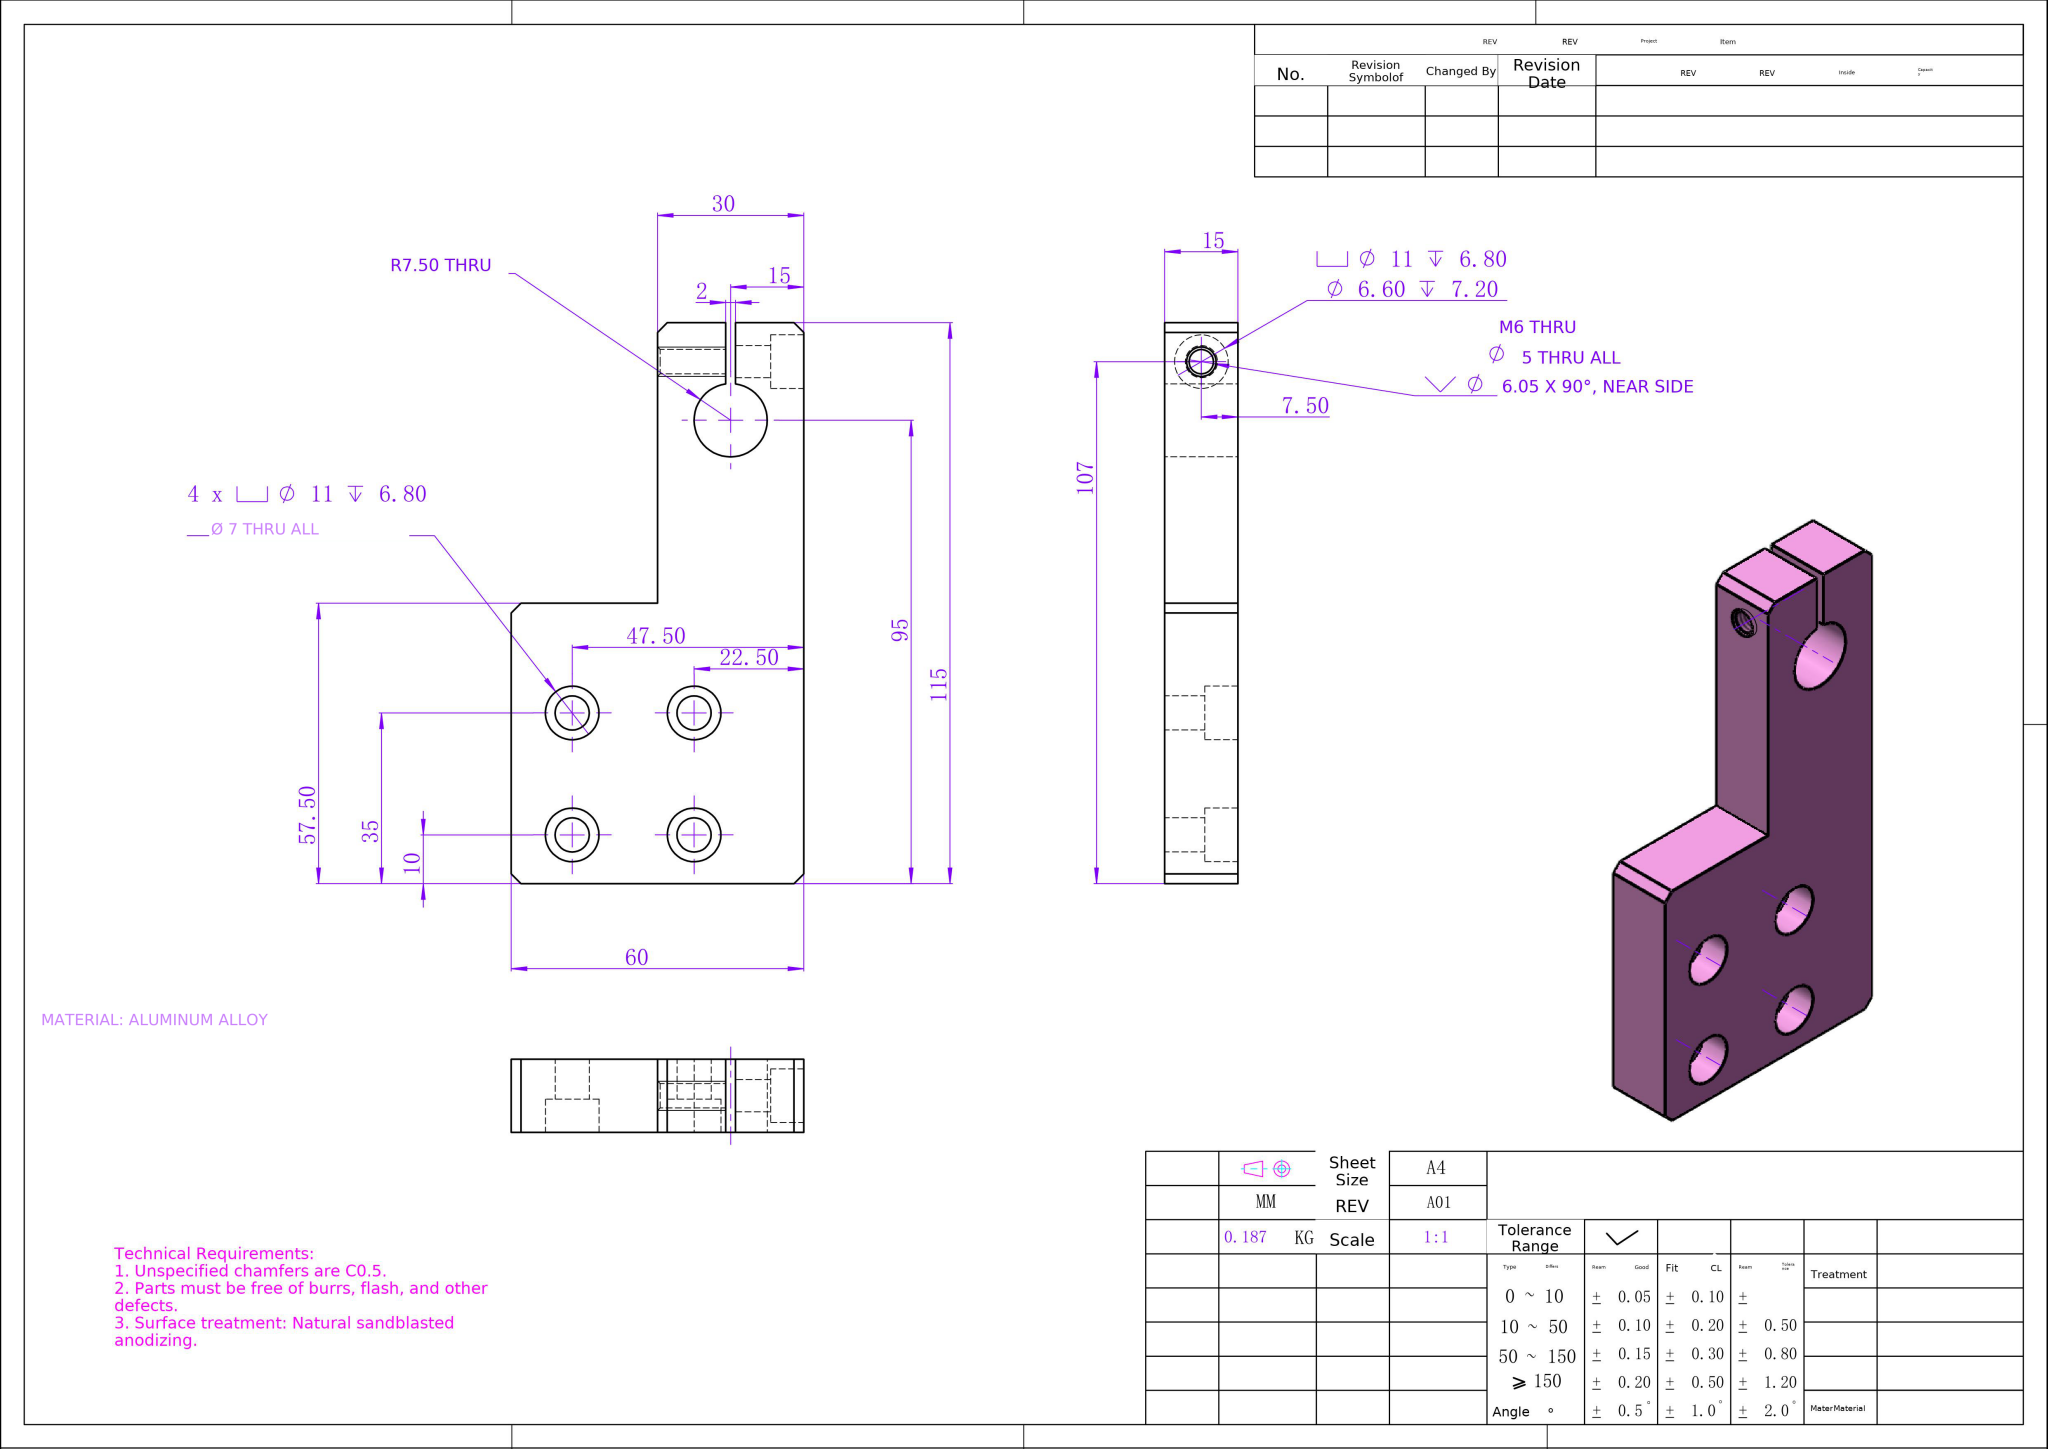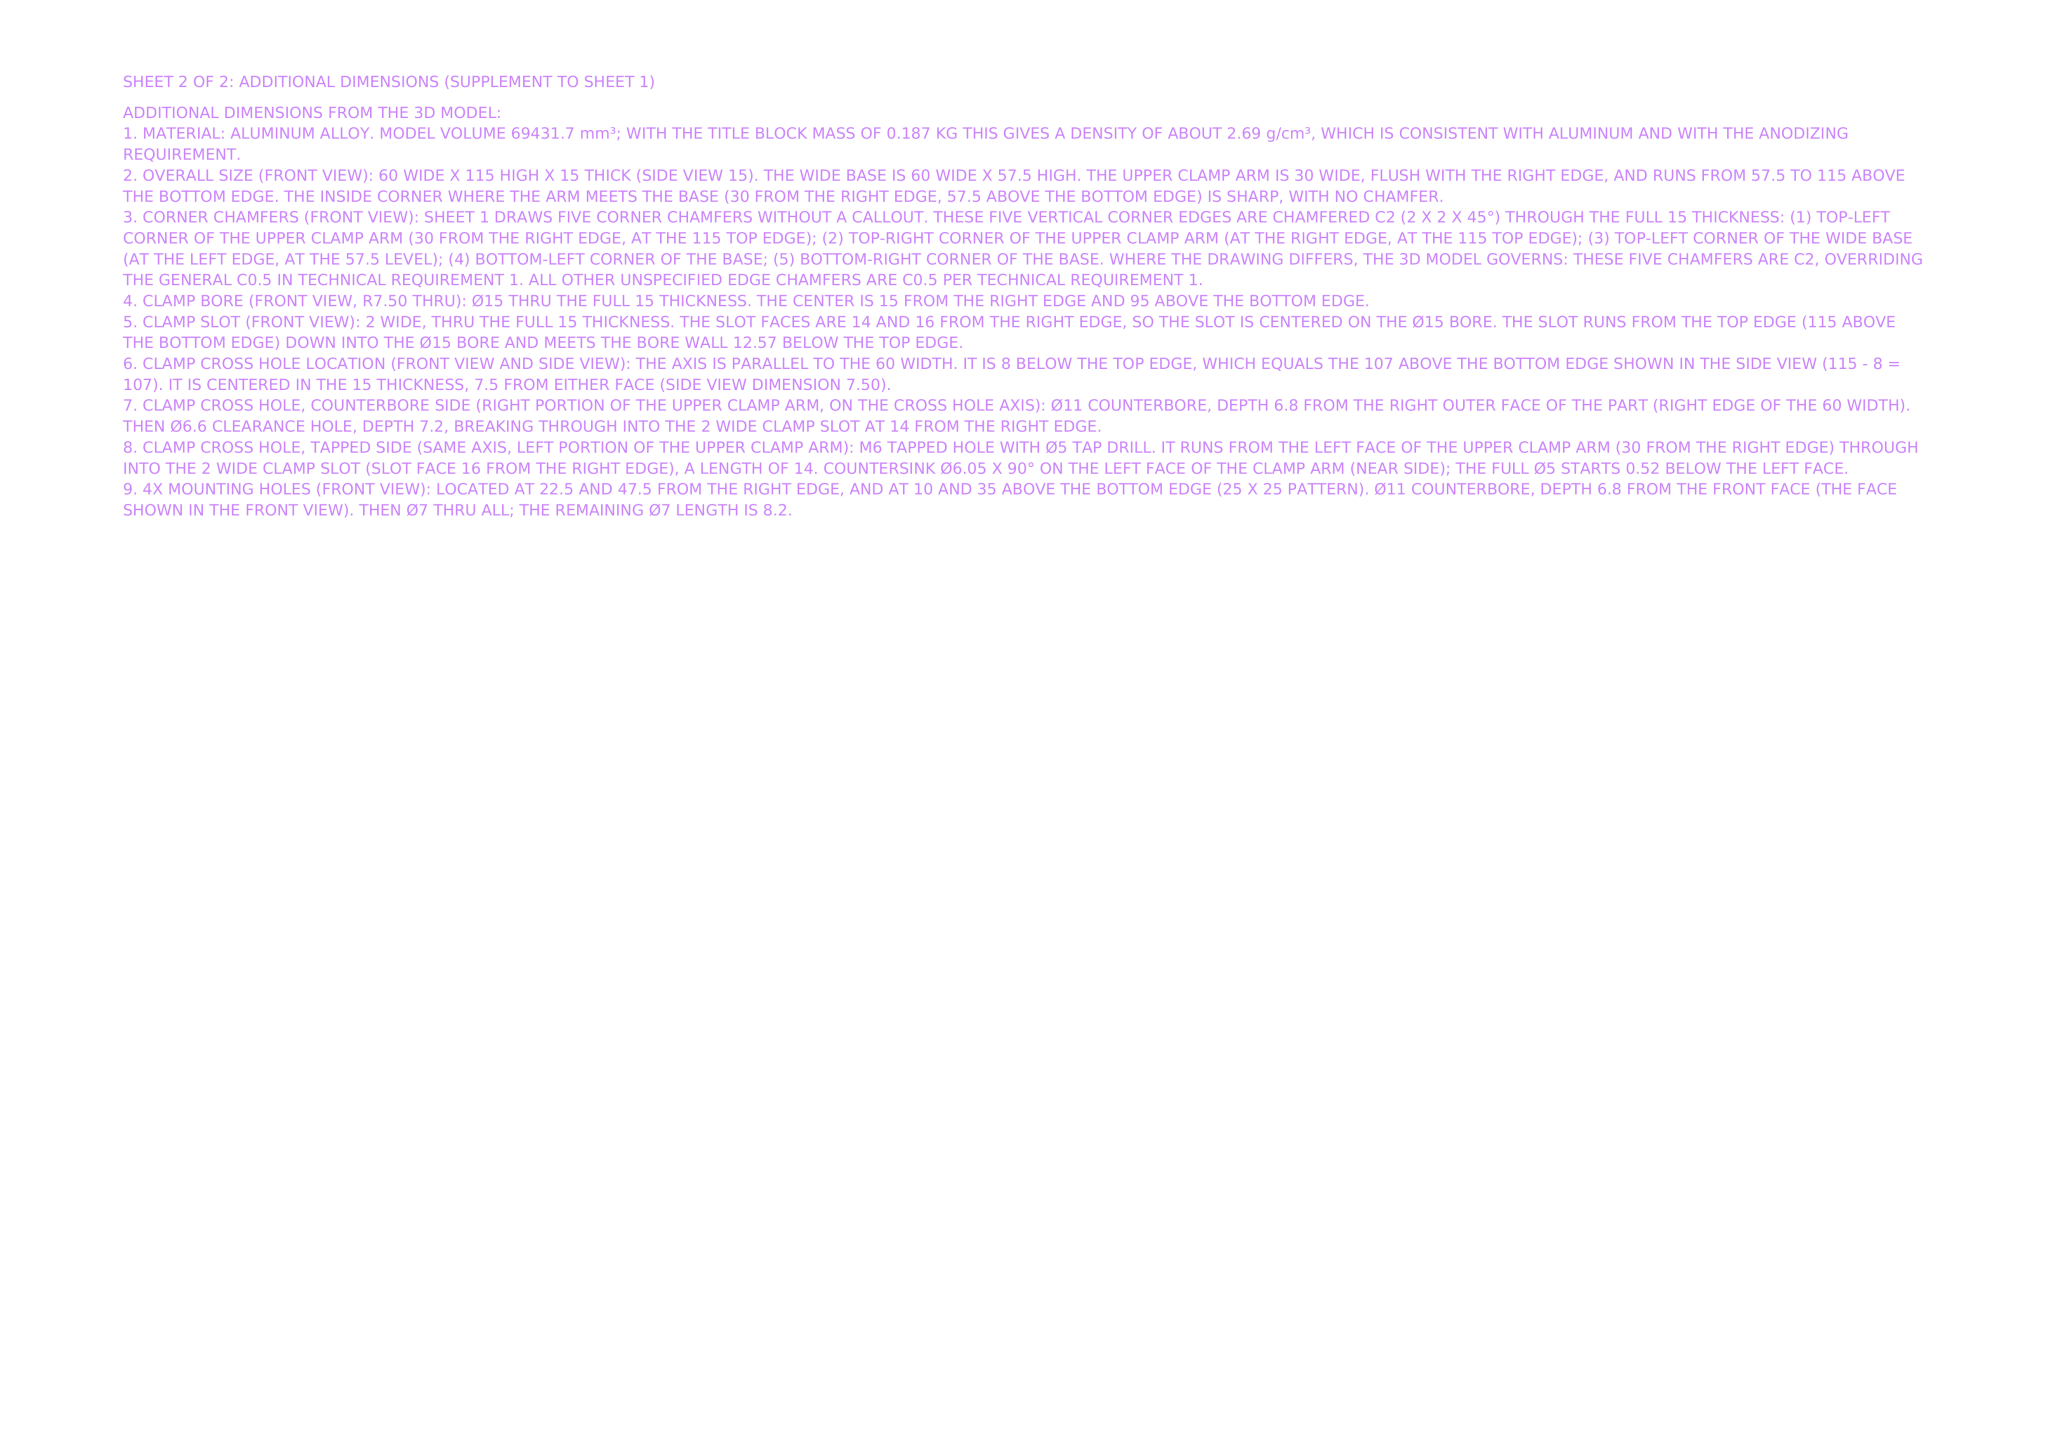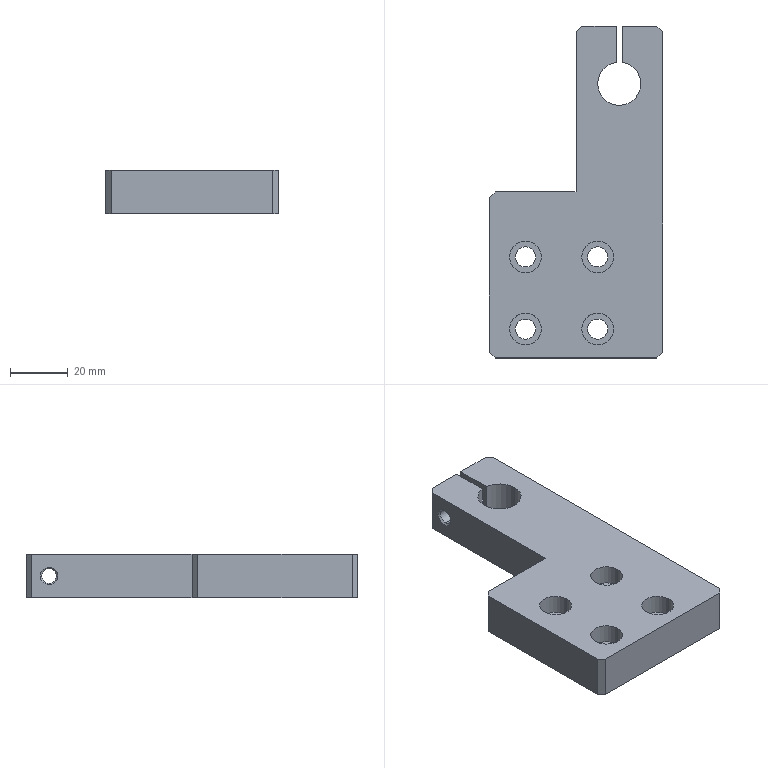Part | NX | mm | 1 solid | 48 faces | box 60 x 115 x 15 mm | volume 69432 mm3 | cylinder 25 | plane 21 | cone 2 | commonest cylinder face diameters 11 x10 7 x8 15 x3 5 x2 6.6 x2